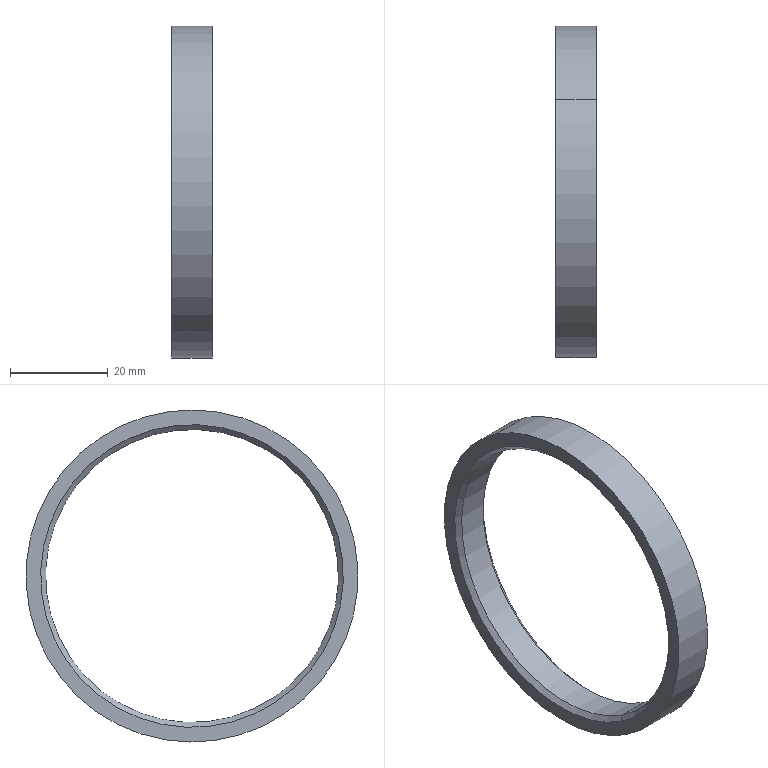Component | SolidWorks | SpindleSleeve2-1 | 1 solid | 10 faces | box 8.25 x 68 x 68 mm | volume 6444 mm3 | cone 4 | cylinder 4 | plane 2 | commonest cylinder face diameters 60 x2 68 x2
build123d program:
from build123d import *

# Parameters (mm, degrees)
SKETCH1_R           = 34
SKETCH1_R_2         = 30
BOSS_EXTRUDE1_DEPTH = 4.125
CHAMFER1_SIZE       = 1


with BuildPart() as part:
    # Sketch1 → Boss-Extrude1 (new, symmetric)
    with BuildSketch(Plane(origin=(0, 0, 0), x_dir=(1, 0, 0), z_dir=(0, 1, 0))):
        with Locations(Location((0, 0, 0), (0, 0, 270))):
            Circle(SKETCH1_R)
        with Locations(Location((0, 0, 0), (0, 0, 270))):
            Circle(SKETCH1_R_2, mode=Mode.SUBTRACT)
    extrude(amount=BOSS_EXTRUDE1_DEPTH, both=True)

    # Chamfer1
    chamfer1_edges = [part.edges().sort_by_distance(p)[0] for p in [
        (0, -4.125, -30),
        (0, 4.125, -30),
    ]]
    chamfer(chamfer1_edges, length=CHAMFER1_SIZE)


solid = part.part

# Placed as in the assembly
solid = solid.moved(Location((538.678, 34.532, 0), (0, 0, 90)))
STEP:
#1=COLOUR_RGB('',0.7922,0.8196,0.9333);
#2=FILL_AREA_STYLE_COLOUR('',#1);
#3=FILL_AREA_STYLE('',(#2));
#4=SURFACE_STYLE_FILL_AREA(#3);
#5=SURFACE_SIDE_STYLE('',(#4));
#6=SURFACE_STYLE_USAGE(.BOTH.,#5);
#7=PRESENTATION_STYLE_ASSIGNMENT((#6));
#8=CARTESIAN_POINT('',(21.085,2.013,0.9842));
#9=VERTEX_POINT('',#8);
#10=CARTESIAN_POINT('',(21.085,0.7065,-0.9842));
#11=VERTEX_POINT('',#10);
#12=CARTESIAN_POINT('',(21.085,1.36,0.));
#13=DIRECTION('',(-1.,0.,0.));
#14=DIRECTION('',(0.,-0.5529,-0.8333));
#15=AXIS2_PLACEMENT_3D('',#12,#13,#14);
#16=CIRCLE('',#15,1.181);
#17=EDGE_CURVE('',#9,#11,#16,.T.);
#18=ORIENTED_EDGE('',*,*,#17,.F.);
#19=CARTESIAN_POINT('',(21.045,2.034,1.017));
#20=VERTEX_POINT('',#19);
#21=CARTESIAN_POINT('',(21.085,2.013,0.9842));
#22=DIRECTION('',(-0.7071,0.3909,0.5892));
#23=VECTOR('',#22,39.37);
#24=LINE('',#21,#23);
#25=EDGE_CURVE('',#9,#20,#24,.T.);
#26=ORIENTED_EDGE('',*,*,#25,.T.);
#27=CARTESIAN_POINT('',(21.045,0.6848,-1.017));
#28=VERTEX_POINT('',#27);
#29=CARTESIAN_POINT('',(21.045,1.36,0.));
#30=DIRECTION('',(1.,0.,0.));
#31=DIRECTION('',(0.,-0.5529,-0.8333));
#32=AXIS2_PLACEMENT_3D('',#29,#30,#31);
#33=CIRCLE('',#32,1.22);
#34=EDGE_CURVE('',#28,#20,#33,.T.);
#35=ORIENTED_EDGE('',*,*,#34,.F.);
#36=CARTESIAN_POINT('',(21.085,0.7065,-0.9842));
#37=DIRECTION('',(-0.7071,-0.3909,-0.5892));
#38=VECTOR('',#37,39.37);
#39=LINE('',#36,#38);
#40=EDGE_CURVE('',#11,#28,#39,.T.);
#41=ORIENTED_EDGE('',*,*,#40,.F.);
#42=EDGE_LOOP('',(#18,#26,#35,#41));
#43=FACE_OUTER_BOUND('',#42,.T.);
#44=CARTESIAN_POINT('',(21.085,1.36,0.));
#45=DIRECTION('',(-1.,0.,0.));
#46=DIRECTION('',(0.,-0.5529,-0.8333));
#47=AXIS2_PLACEMENT_3D('',#44,#45,#46);
#48=CONICAL_SURFACE('',#47,1.181,0.7854);
#49=ADVANCED_FACE('',(#43),#48,.F.);
#50=CARTESIAN_POINT('',(21.331,0.7065,-0.9842));
#51=VERTEX_POINT('',#50);
#52=CARTESIAN_POINT('',(21.331,2.013,0.9842));
#53=VERTEX_POINT('',#52);
#54=CARTESIAN_POINT('',(21.331,1.36,0.));
#55=DIRECTION('',(1.,0.,0.));
#56=DIRECTION('',(0.,-0.5529,-0.8333));
#57=AXIS2_PLACEMENT_3D('',#54,#55,#56);
#58=CIRCLE('',#57,1.181);
#59=EDGE_CURVE('',#51,#53,#58,.T.);
#60=ORIENTED_EDGE('',*,*,#59,.F.);
#61=CARTESIAN_POINT('',(21.37,0.6848,-1.017));
#62=VERTEX_POINT('',#61);
#63=CARTESIAN_POINT('',(21.37,0.6848,-1.017));
#64=DIRECTION('',(0.7071,-0.3909,-0.5892));
#65=VECTOR('',#64,39.37);
#66=LINE('',#63,#65);
#67=EDGE_CURVE('',#51,#62,#66,.T.);
#68=ORIENTED_EDGE('',*,*,#67,.T.);
#69=CARTESIAN_POINT('',(21.37,2.034,1.017));
#70=VERTEX_POINT('',#69);
#71=CARTESIAN_POINT('',(21.37,1.36,0.));
#72=DIRECTION('',(-1.,0.,0.));
#73=DIRECTION('',(0.,-0.5529,-0.8333));
#74=AXIS2_PLACEMENT_3D('',#71,#72,#73);
#75=CIRCLE('',#74,1.22);
#76=EDGE_CURVE('',#70,#62,#75,.T.);
#77=ORIENTED_EDGE('',*,*,#76,.F.);
#78=CARTESIAN_POINT('',(21.37,2.034,1.017));
#79=DIRECTION('',(0.7071,0.3909,0.5892));
#80=VECTOR('',#79,39.37);
#81=LINE('',#78,#80);
#82=EDGE_CURVE('',#53,#70,#81,.T.);
#83=ORIENTED_EDGE('',*,*,#82,.F.);
#84=EDGE_LOOP('',(#60,#68,#77,#83));
#85=FACE_OUTER_BOUND('',#84,.T.);
#86=CARTESIAN_POINT('',(21.37,1.36,0.));
#87=DIRECTION('',(1.,0.,0.));
#88=DIRECTION('',(0.,0.5529,0.8333));
#89=AXIS2_PLACEMENT_3D('',#86,#87,#88);
#90=CONICAL_SURFACE('',#89,1.22,0.7854);
#91=ADVANCED_FACE('',(#85),#90,.F.);
#92=ORIENTED_EDGE('',*,*,#17,.T.);
#93=CARTESIAN_POINT('',(21.045,0.7065,-0.9842));
#94=DIRECTION('',(1.,0.,0.));
#95=VECTOR('',#94,39.37);
#96=LINE('',#93,#95);
#97=EDGE_CURVE('',#11,#51,#96,.T.);
#98=ORIENTED_EDGE('',*,*,#97,.T.);
#99=ORIENTED_EDGE('',*,*,#59,.T.);
#100=CARTESIAN_POINT('',(21.045,2.013,0.9842));
#101=DIRECTION('',(1.,0.,0.));
#102=VECTOR('',#101,39.37);
#103=LINE('',#100,#102);
#104=EDGE_CURVE('',#9,#53,#103,.T.);
#105=ORIENTED_EDGE('',*,*,#104,.F.);
#106=EDGE_LOOP('',(#92,#98,#99,#105));
#107=FACE_OUTER_BOUND('',#106,.T.);
#108=CARTESIAN_POINT('',(21.045,1.36,0.));
#109=DIRECTION('',(1.,0.,0.));
#110=DIRECTION('',(0.,0.5529,0.8333));
#111=AXIS2_PLACEMENT_3D('',#108,#109,#110);
#112=CYLINDRICAL_SURFACE('',#111,1.181);
#113=ADVANCED_FACE('',(#107),#112,.F.);
#114=CARTESIAN_POINT('',(21.045,0.6195,-1.115));
#115=VERTEX_POINT('',#114);
#116=CARTESIAN_POINT('',(21.045,2.1,1.115));
#117=VERTEX_POINT('',#116);
#118=CARTESIAN_POINT('',(21.045,1.36,0.));
#119=DIRECTION('',(-1.,0.,0.));
#120=DIRECTION('',(0.,-0.5529,-0.8333));
#121=AXIS2_PLACEMENT_3D('',#118,#119,#120);
#122=CIRCLE('',#121,1.339);
#123=EDGE_CURVE('',#115,#117,#122,.T.);
#124=ORIENTED_EDGE('',*,*,#123,.F.);
#125=CARTESIAN_POINT('',(21.37,0.6195,-1.115));
#126=VERTEX_POINT('',#125);
#127=CARTESIAN_POINT('',(21.045,0.6195,-1.115));
#128=DIRECTION('',(1.,0.,0.));
#129=VECTOR('',#128,39.37);
#130=LINE('',#127,#129);
#131=EDGE_CURVE('',#115,#126,#130,.T.);
#132=ORIENTED_EDGE('',*,*,#131,.T.);
#133=CARTESIAN_POINT('',(21.37,2.1,1.115));
#134=VERTEX_POINT('',#133);
#135=CARTESIAN_POINT('',(21.37,1.36,0.));
#136=DIRECTION('',(-1.,0.,0.));
#137=DIRECTION('',(0.,-0.5529,-0.8333));
#138=AXIS2_PLACEMENT_3D('',#135,#136,#137);
#139=CIRCLE('',#138,1.339);
#140=EDGE_CURVE('',#126,#134,#139,.T.);
#141=ORIENTED_EDGE('',*,*,#140,.T.);
#142=CARTESIAN_POINT('',(21.045,2.1,1.115));
#143=DIRECTION('',(1.,0.,0.));
#144=VECTOR('',#143,39.37);
#145=LINE('',#142,#144);
#146=EDGE_CURVE('',#117,#134,#145,.T.);
#147=ORIENTED_EDGE('',*,*,#146,.F.);
#148=EDGE_LOOP('',(#124,#132,#141,#147));
#149=FACE_OUTER_BOUND('',#148,.T.);
#150=CARTESIAN_POINT('',(21.045,1.36,0.));
#151=DIRECTION('',(1.,0.,0.));
#152=DIRECTION('',(0.,0.5529,0.8333));
#153=AXIS2_PLACEMENT_3D('',#150,#151,#152);
#154=CYLINDRICAL_SURFACE('',#153,1.339);
#155=ADVANCED_FACE('',(#149),#154,.T.);
#156=ORIENTED_EDGE('',*,*,#34,.T.);
#157=CARTESIAN_POINT('',(21.045,1.36,0.));
#158=DIRECTION('',(1.,0.,0.));
#159=DIRECTION('',(0.,-0.5529,-0.8333));
#160=AXIS2_PLACEMENT_3D('',#157,#158,#159);
#161=CIRCLE('',#160,1.22);
#162=EDGE_CURVE('',#20,#28,#161,.T.);
#163=ORIENTED_EDGE('',*,*,#162,.T.);
#164=EDGE_LOOP('',(#156,#163));
#165=FACE_BOUND('',#164,.T.);
#166=CARTESIAN_POINT('',(21.045,1.36,0.));
#167=DIRECTION('',(-1.,0.,0.));
#168=DIRECTION('',(0.,-0.5529,-0.8333));
#169=AXIS2_PLACEMENT_3D('',#166,#167,#168);
#170=CIRCLE('',#169,1.339);
#171=EDGE_CURVE('',#117,#115,#170,.T.);
#172=ORIENTED_EDGE('',*,*,#171,.T.);
#173=ORIENTED_EDGE('',*,*,#123,.T.);
#174=EDGE_LOOP('',(#172,#173));
#175=FACE_OUTER_BOUND('',#174,.T.);
#176=CARTESIAN_POINT('',(21.045,1.36,0.));
#177=DIRECTION('',(-1.,0.,0.));
#178=DIRECTION('',(0.,-0.5529,-0.8333));
#179=AXIS2_PLACEMENT_3D('',#176,#177,#178);
#180=PLANE('',#179);
#181=ADVANCED_FACE('',(#165,#175),#180,.T.);
#182=ORIENTED_EDGE('',*,*,#76,.T.);
#183=CARTESIAN_POINT('',(21.37,1.36,0.));
#184=DIRECTION('',(-1.,0.,0.));
#185=DIRECTION('',(0.,-0.5529,-0.8333));
#186=AXIS2_PLACEMENT_3D('',#183,#184,#185);
#187=CIRCLE('',#186,1.22);
#188=EDGE_CURVE('',#62,#70,#187,.T.);
#189=ORIENTED_EDGE('',*,*,#188,.T.);
#190=EDGE_LOOP('',(#182,#189));
#191=FACE_BOUND('',#190,.T.);
#192=CARTESIAN_POINT('',(21.37,1.36,0.));
#193=DIRECTION('',(-1.,0.,0.));
#194=DIRECTION('',(0.,-0.5529,-0.8333));
#195=AXIS2_PLACEMENT_3D('',#192,#193,#194);
#196=CIRCLE('',#195,1.339);
#197=EDGE_CURVE('',#134,#126,#196,.T.);
#198=ORIENTED_EDGE('',*,*,#197,.F.);
#199=ORIENTED_EDGE('',*,*,#140,.F.);
#200=EDGE_LOOP('',(#198,#199));
#201=FACE_OUTER_BOUND('',#200,.T.);
#202=CARTESIAN_POINT('',(21.37,1.36,0.));
#203=DIRECTION('',(-1.,0.,0.));
#204=DIRECTION('',(0.,-0.5529,-0.8333));
#205=AXIS2_PLACEMENT_3D('',#202,#203,#204);
#206=PLANE('',#205);
#207=ADVANCED_FACE('',(#191,#201),#206,.F.);
#208=ORIENTED_EDGE('',*,*,#131,.F.);
#209=ORIENTED_EDGE('',*,*,#171,.F.);
#210=ORIENTED_EDGE('',*,*,#146,.T.);
#211=ORIENTED_EDGE('',*,*,#197,.T.);
#212=EDGE_LOOP('',(#208,#209,#210,#211));
#213=FACE_OUTER_BOUND('',#212,.T.);
#214=CARTESIAN_POINT('',(21.045,1.36,0.));
#215=DIRECTION('',(1.,0.,0.));
#216=DIRECTION('',(0.,0.5529,0.8333));
#217=AXIS2_PLACEMENT_3D('',#214,#215,#216);
#218=CYLINDRICAL_SURFACE('',#217,1.339);
#219=ADVANCED_FACE('',(#213),#218,.T.);
#220=ORIENTED_EDGE('',*,*,#97,.F.);
#221=CARTESIAN_POINT('',(21.085,1.36,0.));
#222=DIRECTION('',(-1.,0.,0.));
#223=DIRECTION('',(0.,-0.5529,-0.8333));
#224=AXIS2_PLACEMENT_3D('',#221,#222,#223);
#225=CIRCLE('',#224,1.181);
#226=EDGE_CURVE('',#11,#9,#225,.T.);
#227=ORIENTED_EDGE('',*,*,#226,.T.);
#228=ORIENTED_EDGE('',*,*,#104,.T.);
#229=CARTESIAN_POINT('',(21.331,1.36,0.));
#230=DIRECTION('',(1.,0.,0.));
#231=DIRECTION('',(0.,-0.5529,-0.8333));
#232=AXIS2_PLACEMENT_3D('',#229,#230,#231);
#233=CIRCLE('',#232,1.181);
#234=EDGE_CURVE('',#53,#51,#233,.T.);
#235=ORIENTED_EDGE('',*,*,#234,.T.);
#236=EDGE_LOOP('',(#220,#227,#228,#235));
#237=FACE_OUTER_BOUND('',#236,.T.);
#238=CARTESIAN_POINT('',(21.045,1.36,0.));
#239=DIRECTION('',(1.,0.,0.));
#240=DIRECTION('',(0.,0.5529,0.8333));
#241=AXIS2_PLACEMENT_3D('',#238,#239,#240);
#242=CYLINDRICAL_SURFACE('',#241,1.181);
#243=ADVANCED_FACE('',(#237),#242,.F.);
#244=ORIENTED_EDGE('',*,*,#67,.F.);
#245=ORIENTED_EDGE('',*,*,#234,.F.);
#246=ORIENTED_EDGE('',*,*,#82,.T.);
#247=ORIENTED_EDGE('',*,*,#188,.F.);
#248=EDGE_LOOP('',(#244,#245,#246,#247));
#249=FACE_OUTER_BOUND('',#248,.T.);
#250=CARTESIAN_POINT('',(21.37,1.36,0.));
#251=DIRECTION('',(1.,0.,0.));
#252=DIRECTION('',(0.,0.5529,0.8333));
#253=AXIS2_PLACEMENT_3D('',#250,#251,#252);
#254=CONICAL_SURFACE('',#253,1.22,0.7854);
#255=ADVANCED_FACE('',(#249),#254,.F.);
#256=ORIENTED_EDGE('',*,*,#25,.F.);
#257=ORIENTED_EDGE('',*,*,#226,.F.);
#258=ORIENTED_EDGE('',*,*,#40,.T.);
#259=ORIENTED_EDGE('',*,*,#162,.F.);
#260=EDGE_LOOP('',(#256,#257,#258,#259));
#261=FACE_OUTER_BOUND('',#260,.T.);
#262=CARTESIAN_POINT('',(21.085,1.36,0.));
#263=DIRECTION('',(-1.,0.,0.));
#264=DIRECTION('',(0.,-0.5529,-0.8333));
#265=AXIS2_PLACEMENT_3D('',#262,#263,#264);
#266=CONICAL_SURFACE('',#265,1.181,0.7854);
#267=ADVANCED_FACE('',(#261),#266,.F.);
#268=CLOSED_SHELL('',(#49,#91,#113,#155,#181,#207,#219,#243,#255,#267));
#269=MANIFOLD_SOLID_BREP('',#268);
#270=STYLED_ITEM('',(#7),#269);
#271=(LENGTH_UNIT()NAMED_UNIT(*)SI_UNIT($,.METRE.));
#272=LENGTH_MEASURE_WITH_UNIT(LENGTH_MEASURE(0.0254),#271);
#273=DIMENSIONAL_EXPONENTS(1.,0.,0.,0.,0.,0.,0.);
#274=(CONVERSION_BASED_UNIT('',#272)LENGTH_UNIT()NAMED_UNIT(#273));
#275=UNCERTAINTY_MEASURE_WITH_UNIT(LENGTH_MEASURE(0.00001),#274,'','');
#276=(NAMED_UNIT(*)PLANE_ANGLE_UNIT()SI_UNIT($,.RADIAN.));
#277=(NAMED_UNIT(*)SI_UNIT($,.STERADIAN.)SOLID_ANGLE_UNIT());
#278=(GEOMETRIC_REPRESENTATION_CONTEXT(3)GLOBAL_UNCERTAINTY_ASSIGNED_CONTEXT((#275))GLOBAL_UNIT_ASSIGNED_CONTEXT((#274,#276,#277))REPRESENTATION_CONTEXT('',''));
#279=MECHANICAL_DESIGN_GEOMETRIC_PRESENTATION_REPRESENTATION('',(#270),#278);
#280=PRESENTATION_LAYER_ASSIGNMENT('','',(#270));
#281=CARTESIAN_POINT('',(0.,0.,0.));
#282=DIRECTION('',(0.,0.,1.));
#283=DIRECTION('',(1.,0.,0.));
#284=AXIS2_PLACEMENT_3D('',#281,#282,#283);
#285=(LENGTH_UNIT()NAMED_UNIT(*)SI_UNIT($,.METRE.));
#286=LENGTH_MEASURE_WITH_UNIT(LENGTH_MEASURE(0.0254),#285);
#287=DIMENSIONAL_EXPONENTS(1.,0.,0.,0.,0.,0.,0.);
#288=(CONVERSION_BASED_UNIT('',#286)LENGTH_UNIT()NAMED_UNIT(#287));
#289=UNCERTAINTY_MEASURE_WITH_UNIT(LENGTH_MEASURE(0.00001),#288,'','');
#290=(NAMED_UNIT(*)PLANE_ANGLE_UNIT()SI_UNIT($,.RADIAN.));
#291=(NAMED_UNIT(*)SI_UNIT($,.STERADIAN.)SOLID_ANGLE_UNIT());
#292=(GEOMETRIC_REPRESENTATION_CONTEXT(3)GLOBAL_UNCERTAINTY_ASSIGNED_CONTEXT((#289))GLOBAL_UNIT_ASSIGNED_CONTEXT((#288,#290,#291))REPRESENTATION_CONTEXT('',''));
#293=ADVANCED_BREP_SHAPE_REPRESENTATION('',(#269,#284),#292);